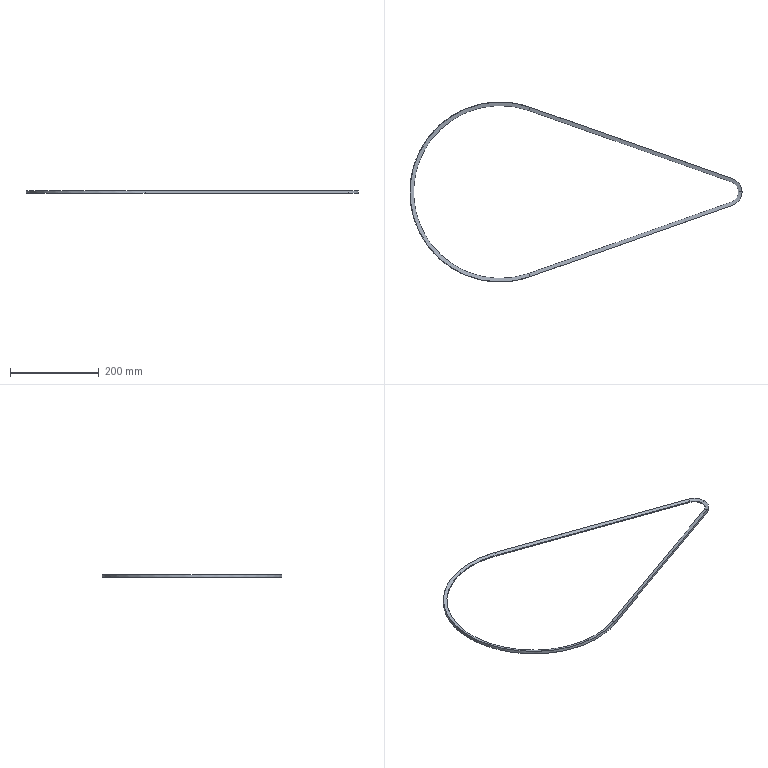Component | SolidWorks | Belt-1 | 1 solid | 22 faces | box 749 x 406 x 6.5 mm | volume 63032 mm3 | plane 10 | cone 6 | cylinder 6 | commonest cylinder face diameters 48 x2 64 x2 406 x1 390 x1
build123d program:
from build123d import *
from OCP.BRepFilletAPI import BRepFilletAPI_MakeChamfer

# Parameters (mm, degrees)
BOSS_EXTRUDE1_DEPTH = 6.5
CHAMFER1_SIZE       = 2.14
CHAMFER1_SIZE2      = 7.96
CHAMFER3_SIZE       = 7.96
CHAMFER3_SIZE2      = 2.14


with BuildPart() as part:
    # Sketch1 → Boss-Extrude1 (new body)
    with BuildSketch(Plane(origin=(0, 0, 0), x_dir=(0, 0, -1), z_dir=(1, 0, 0))):
        with BuildLine():
            Line((-10.646, 30.177), (446.465, 191.437))
            ThreePointArc((446.465, 191.437), (717, 0), (446.465, -191.437))
            Line((446.465, -191.437), (-10.646, -30.177))
            ThreePointArc((-10.646, -30.177), (-32, 0), (-10.646, 30.177))
        make_face()
        with BuildLine():
            Line((-7.984, 22.633), (449.126, 183.892))
            ThreePointArc((449.126, 183.892), (709, 0), (449.126, -183.892))
            Line((449.126, -183.892), (-7.984, -22.633))
            ThreePointArc((-7.984, -22.633), (-24, 0), (-7.984, 22.633))
        make_face(mode=Mode.SUBTRACT)
    extrude(amount=BOSS_EXTRUDE1_DEPTH)

    # Chamfer1: one chamfer whose edges measure the first distance from different faces: ONE call of the kernel's chamfer builder (chamfer() names one face for all edges)
    chamfer1_edges_1 = [part.edges().sort_by_distance(p)[0] for p in [
        (0, 0, -709),
    ]]
    chamfer1_side_1 = [part.faces().sort_by_distance(p)[0] for p in [
        (3.25, 0, -709),
    ]]
    chamfer1_edges_2 = [part.edges().sort_by_distance(p)[0] for p in [
        (0, 103.263, -220.571),
    ]]
    chamfer1_side_2 = [part.faces().sort_by_distance(p)[0] for p in [
        (3.25, 103.263, -220.571),
    ]]
    chamfer1_edges_3 = [part.edges().sort_by_distance(p)[0] for p in [
        (0, 0, 24),
    ]]
    chamfer1_side_3 = [part.faces().sort_by_distance(p)[0] for p in [
        (3.25, 0, 24),
    ]]
    chamfer1_edges_4 = [part.edges().sort_by_distance(p)[0] for p in [
        (0, -103.263, -220.571),
    ]]
    chamfer1_side_4 = [part.faces().sort_by_distance(p)[0] for p in [
        (3.25, -103.263, -220.571),
    ]]
    chamfer1 = BRepFilletAPI_MakeChamfer(part.part.solid().wrapped)
    for e in chamfer1_edges_1:
        chamfer1.Add(CHAMFER1_SIZE, CHAMFER1_SIZE2, e.wrapped, chamfer1_side_1[0].wrapped)  # the first distance lies on this face
    for e in chamfer1_edges_2:
        chamfer1.Add(CHAMFER1_SIZE, CHAMFER1_SIZE2, e.wrapped, chamfer1_side_2[0].wrapped)  # the first distance lies on this face
    for e in chamfer1_edges_3:
        chamfer1.Add(CHAMFER1_SIZE, CHAMFER1_SIZE2, e.wrapped, chamfer1_side_3[0].wrapped)  # the first distance lies on this face
    for e in chamfer1_edges_4:
        chamfer1.Add(CHAMFER1_SIZE, CHAMFER1_SIZE2, e.wrapped, chamfer1_side_4[0].wrapped)  # the first distance lies on this face
    add(Compound.cast(chamfer1.Shape()), mode=Mode.REPLACE)

    # Chamfer3
    chamfer3_edges = [part.edges().sort_by_distance(p)[0] for p in [
        (6.5, 0, -709),
        (6.5, 103.263, -220.571),
        (6.5, 0, 24),
        (6.5, -103.263, -220.571),
    ]]
    chamfer3_side = [part.faces().sort_by_distance(p)[0] for p in [
        (6.5, 110.004, -218.193),
    ]]
    chamfer(chamfer3_edges, length=CHAMFER3_SIZE, length2=CHAMFER3_SIZE2, reference=chamfer3_side[0])


solid = part.part

# Placed as in the assembly
solid = solid.moved(Location((549.733, 15.31, 118.482), (0, 90, 0)))